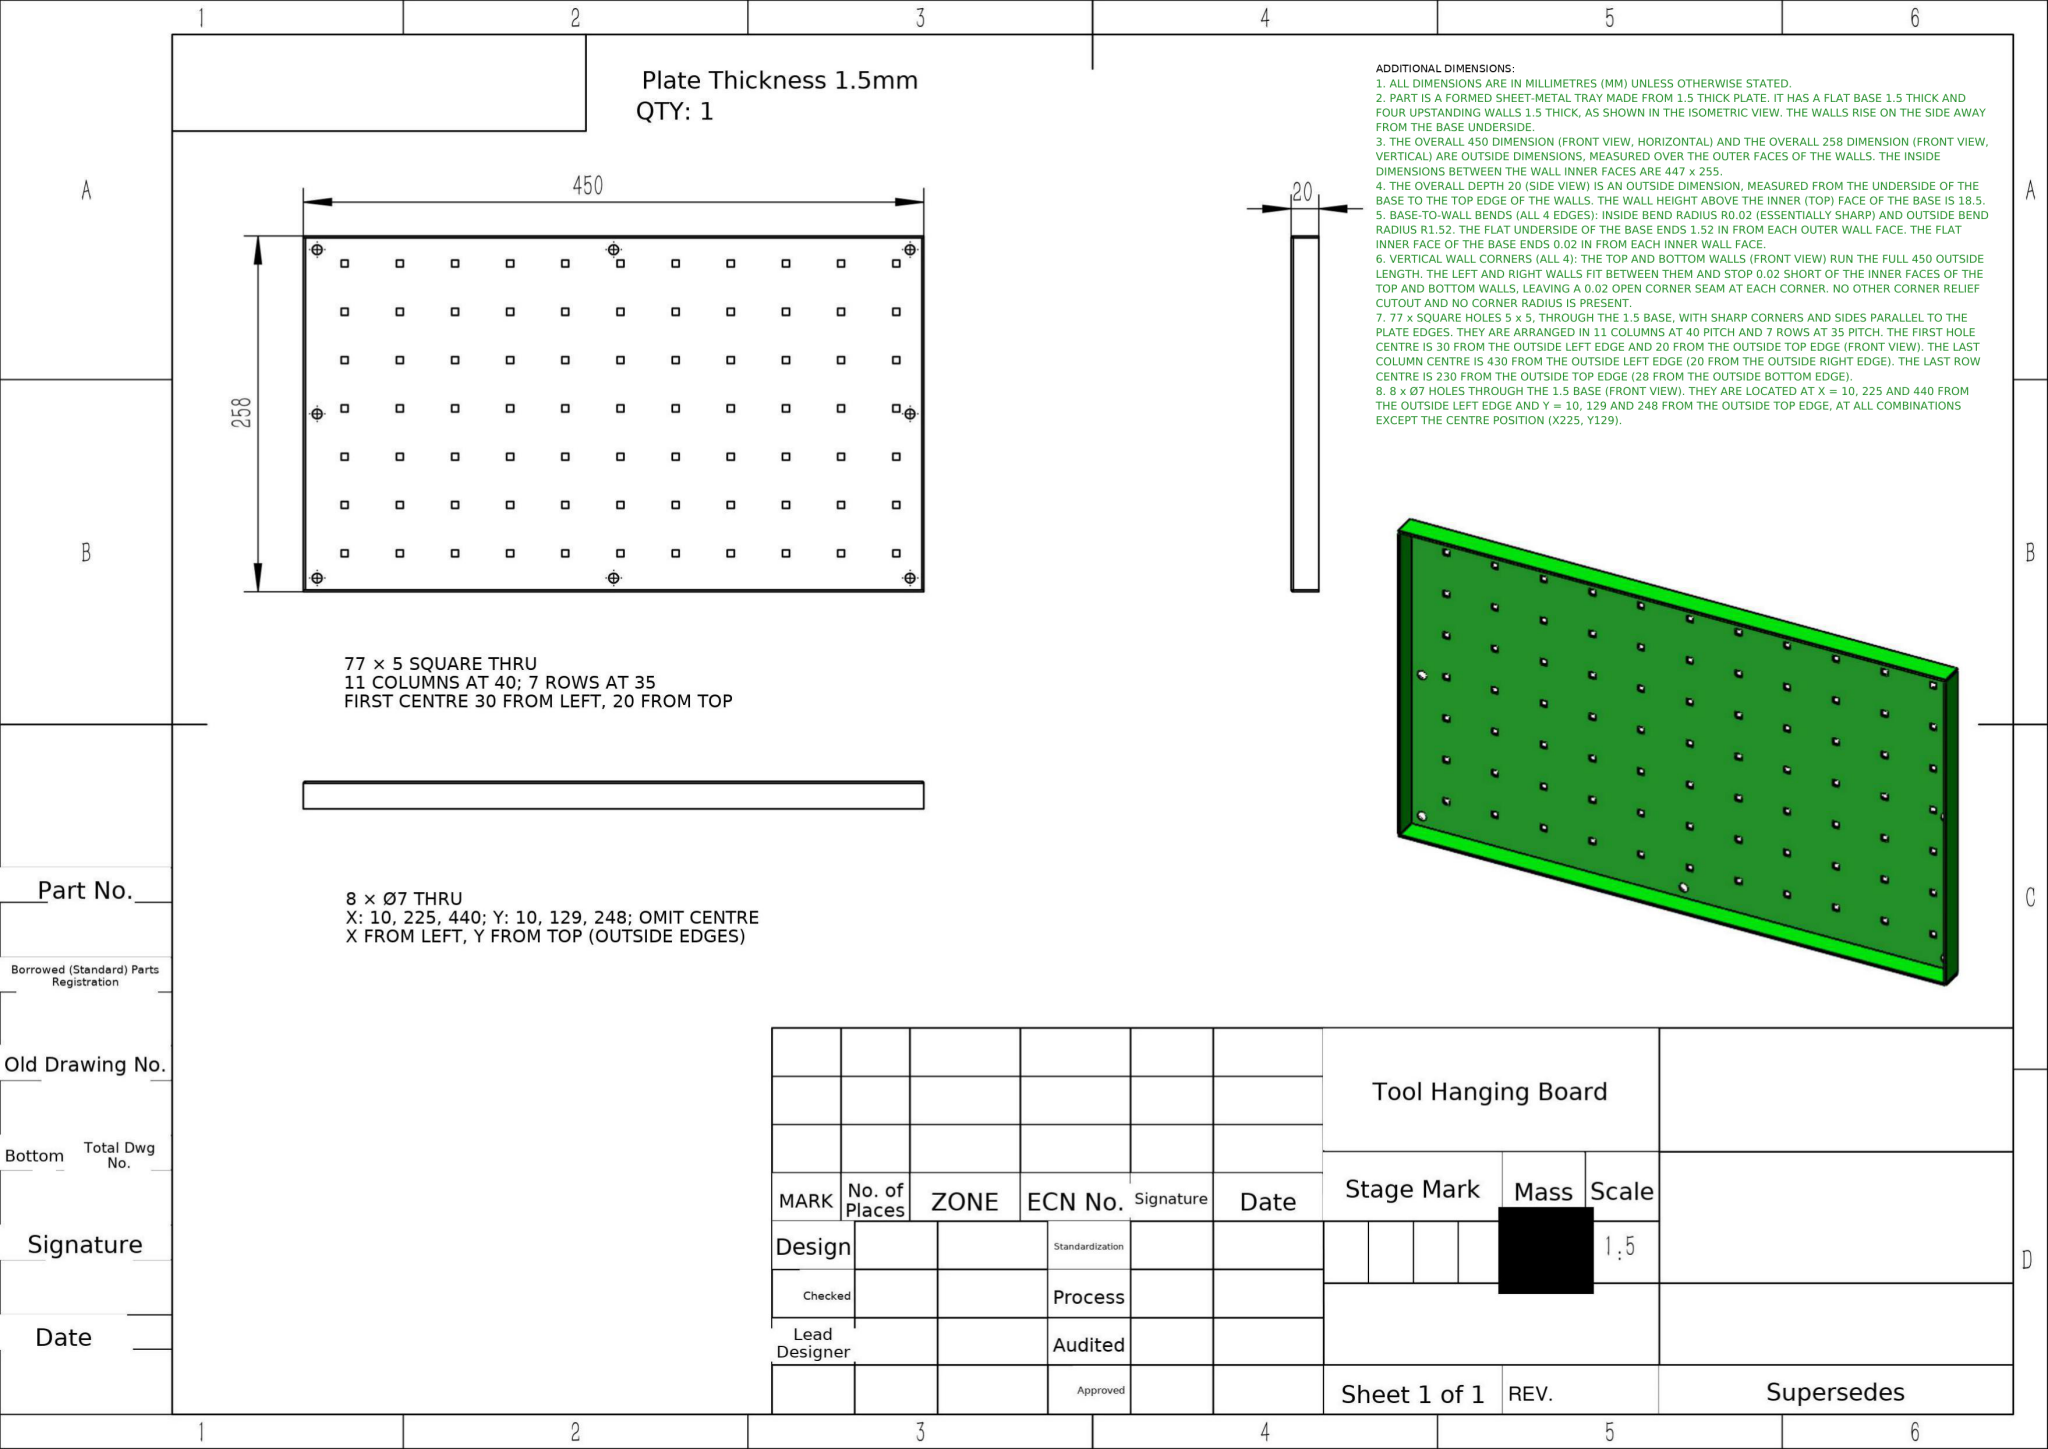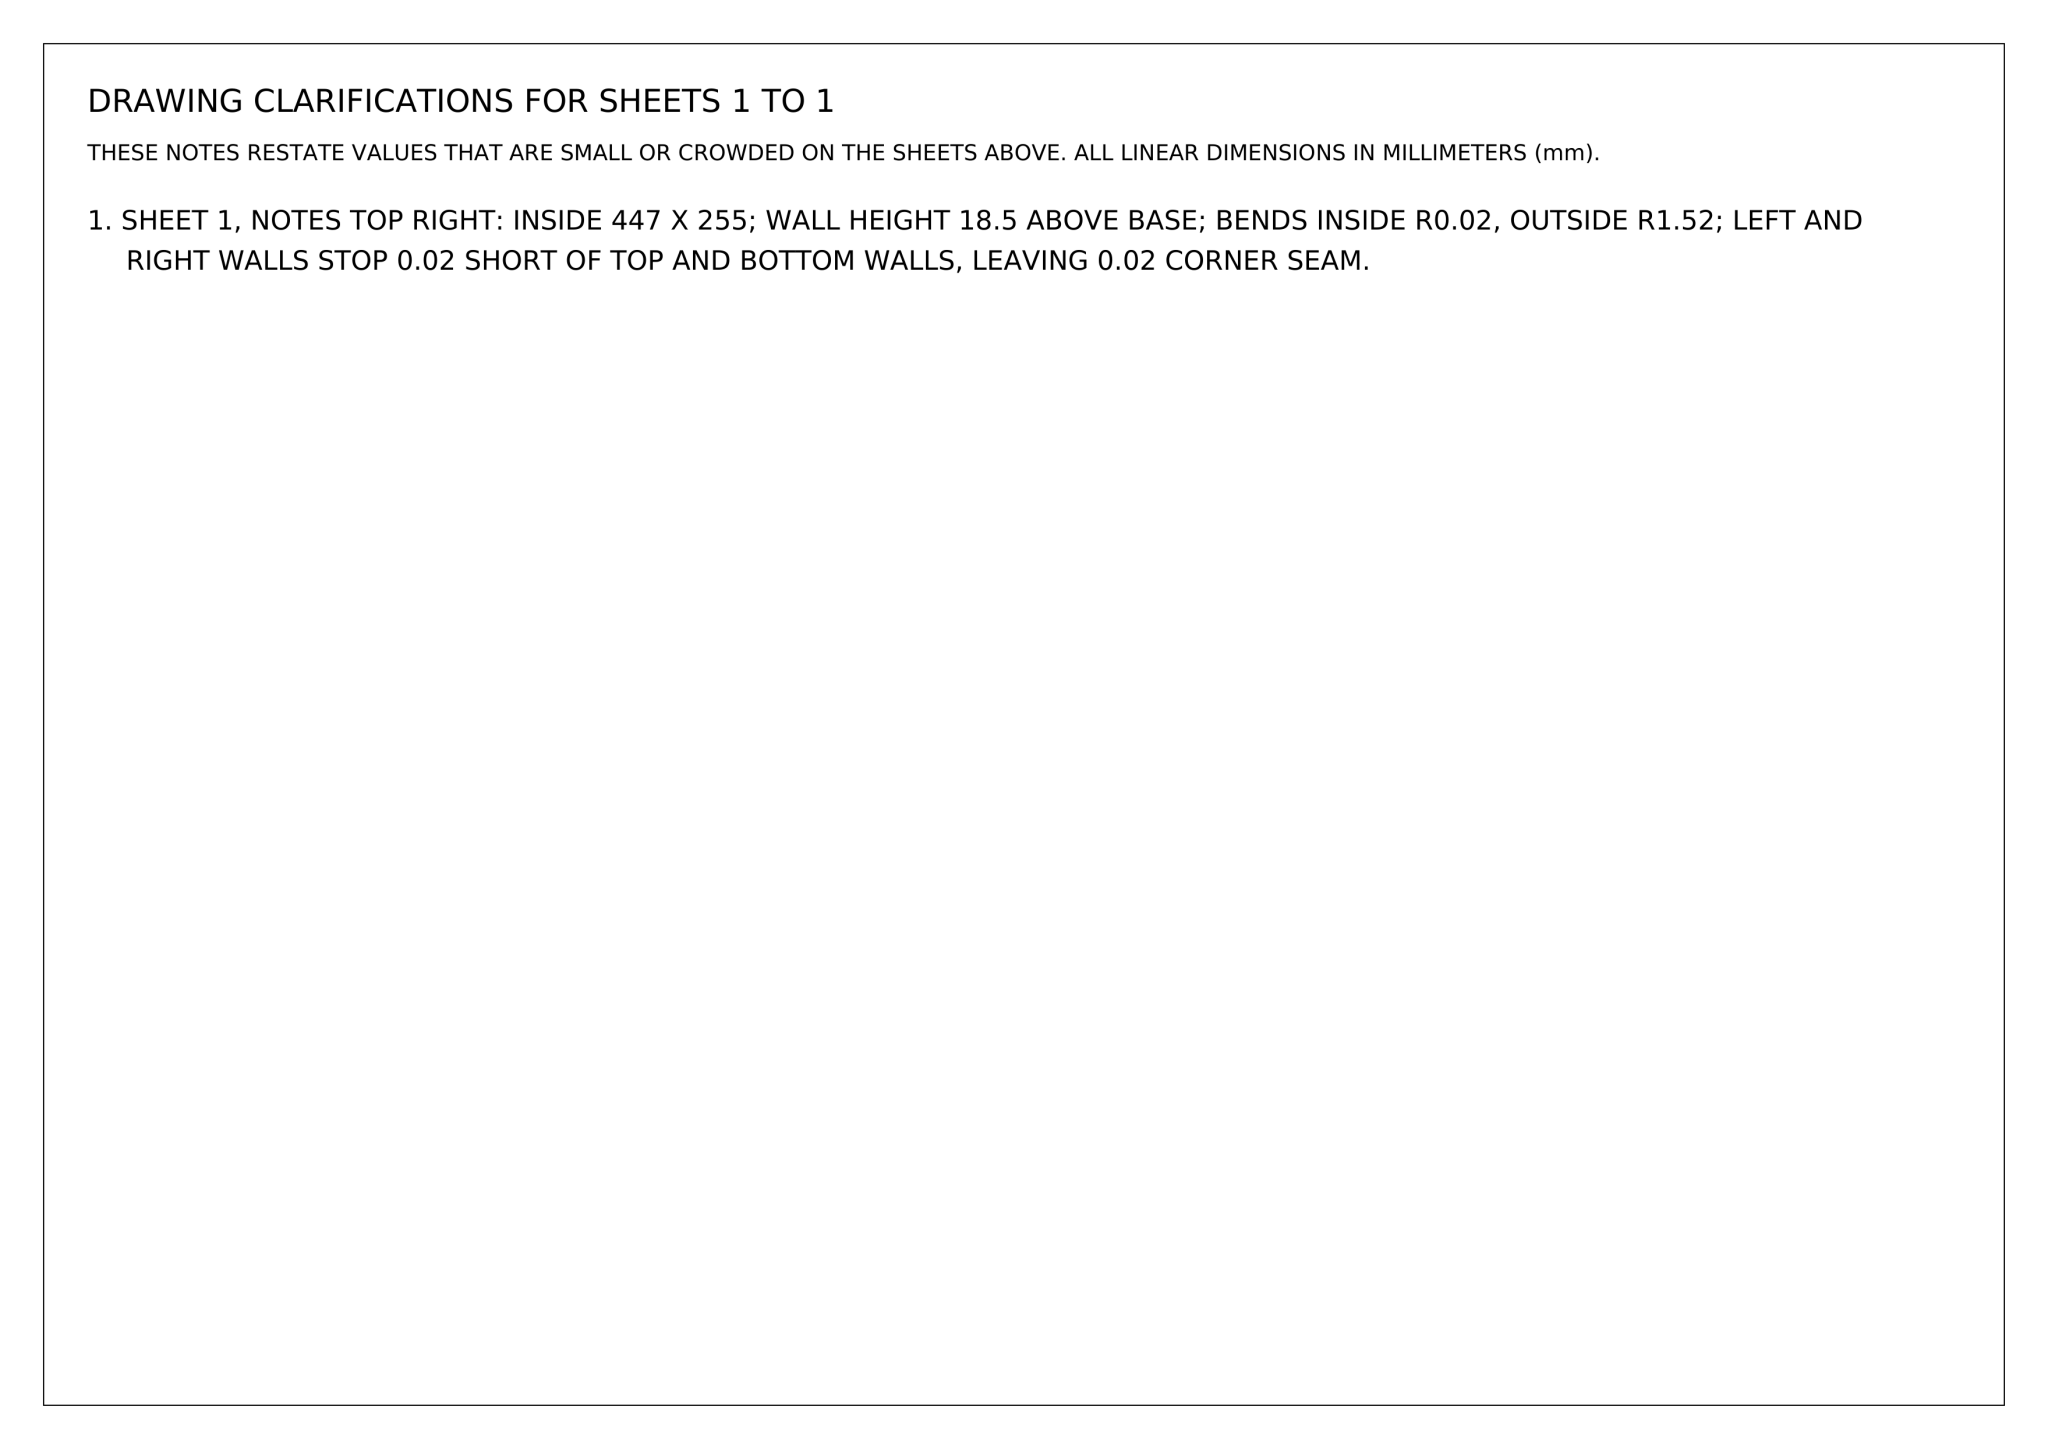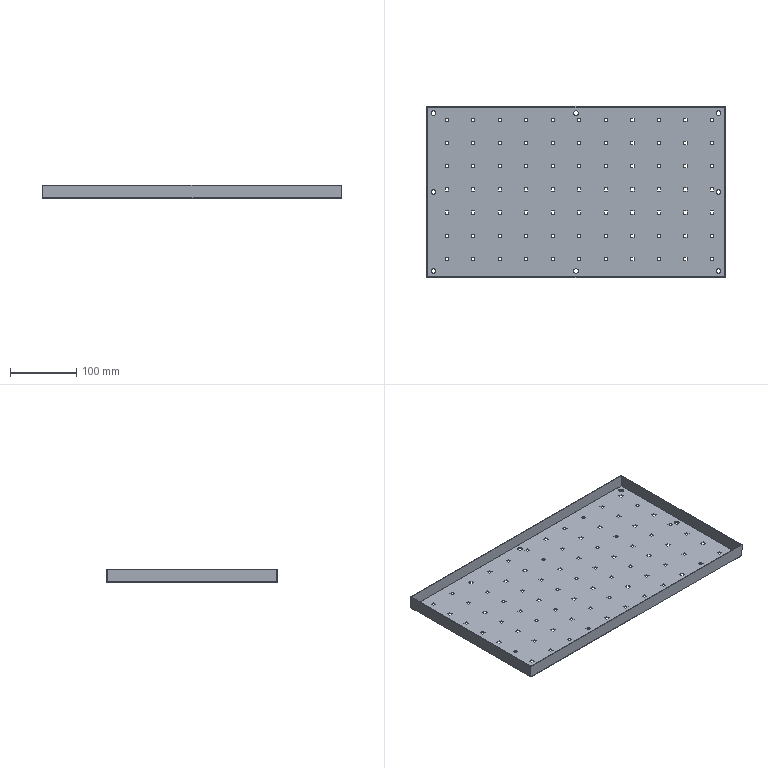Part | NX | mm | Rimmed Perforated Fixture Plate | 1 solid | 366 faces | box 450 x 258 x 20 mm | volume 209216 mm3 | plane 342 | cylinder 24 | commonest cylinder face diameters 7 x16 3.04 x4 0.04 x4